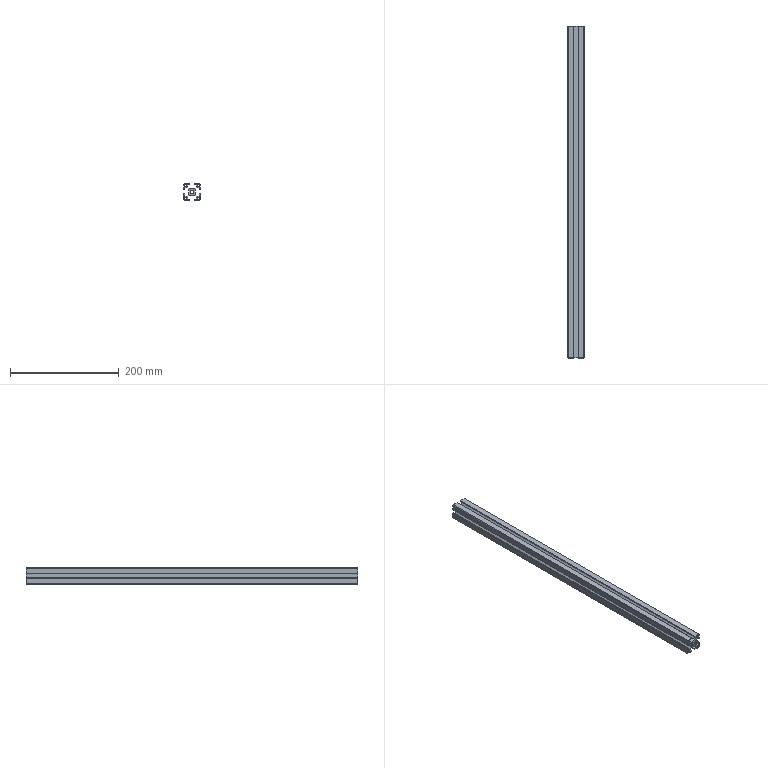Component | SolidWorks | 3030-610-1 | 1 solid | 64 faces | box 30 x 610 x 30 mm | volume 204135 mm3 | plane 46 | cylinder 18 | commonest cylinder face diameters 4.2 x8 0.6 x4 4 x4 6.8 x2
build123d program:
from build123d import *

# Parameters (mm, degrees)
SKETCH1_R           = 2.1
SKETCH1_R_2         = 3.4
BOSS_EXTRUDE1_DEPTH = 610


with BuildPart() as part:
    # Sketch1 → Boss-Extrude1 (new body)
    with BuildSketch(Plane(origin=(0, 0, -100), x_dir=(-1, 0, 0), z_dir=(0, 0, -1))):
        with BuildLine():
            Line((15, 3.8), (15, 13.5))
            ThreePointArc((15, 13.5), (14.823, 14.323), (14.323, 15))
            Line((14.323, 15), (4, 15))
            Line((4, 15), (4, 13))
            Line((4, 13), (8.25, 13))
            Line((8.25, 13), (8.25, 9.664))
            Line((8.25, 9.664), (4.586, 6))
            Line((4.586, 6), (-4.586, 6))
            Line((-4.586, 6), (-8.25, 9.664))
            Line((-8.25, 9.664), (-8.25, 13))
            Line((-8.25, 13), (-4, 13))
            Line((-4, 13), (-4, 15))
            Line((-4, 15), (-14.323, 15))
            ThreePointArc((-14.323, 15), (-14.823, 14.323), (-15, 13.5))
            Line((-15, 13.5), (-15, 3.8))
            ThreePointArc((-15, 3.8), (-14.912, 3.588), (-14.7, 3.5))
            Line((-14.7, 3.5), (-13, 3.5))
            Line((-13, 3.5), (-13, 8.25))
            Line((-13, 8.25), (-9.664, 8.25))
            Line((-9.664, 8.25), (-6, 4.586))
            Line((-6, 4.586), (-6, -4.586))
            Line((-6, -4.586), (-9.664, -8.25))
            Line((-9.664, -8.25), (-13, -8.25))
            Line((-13, -8.25), (-13, -4.5))
            Line((-13, -4.5), (-14.7, -4.5))
            ThreePointArc((-14.7, -4.5), (-14.912, -4.588), (-15, -4.8))
            Line((-15, -4.8), (-15, -13.5))
            ThreePointArc((-15, -13.5), (-14.823, -14.323), (-14.323, -15))
            Line((-14.323, -15), (-4, -15))
            Line((-4, -15), (-4, -13))
            Line((-4, -13), (-8.25, -13))
            Line((-8.25, -13), (-8.25, -9.664))
            Line((-8.25, -9.664), (-4.586, -6))
            Line((-4.586, -6), (4.586, -6))
            Line((4.586, -6), (8.25, -9.664))
            Line((8.25, -9.664), (8.25, -13))
            Line((8.25, -13), (4, -13))
            Line((4, -13), (4, -15))
            Line((4, -15), (14.323, -15))
            ThreePointArc((14.323, -15), (14.823, -14.323), (15, -13.5))
            Line((15, -13.5), (15, -4.8))
            ThreePointArc((15, -4.8), (14.912, -4.588), (14.7, -4.5))
            Line((14.7, -4.5), (13, -4.5))
            Line((13, -4.5), (13, -8.25))
            Line((13, -8.25), (9.664, -8.25))
            Line((9.664, -8.25), (6, -4.586))
            Line((6, -4.586), (6, 4.586))
            Line((6, 4.586), (9.664, 8.25))
            Line((9.664, 8.25), (13, 8.25))
            Line((13, 8.25), (13, 3.5))
            Line((13, 3.5), (14.7, 3.5))
            ThreePointArc((14.7, 3.5), (14.912, 3.588), (15, 3.8))
        make_face()
        with Locations(Location((11.625, 11.625, 0), (0, 0, 180))):
            Circle(SKETCH1_R, mode=Mode.SUBTRACT)
        with Locations(Location((11.625, -11.625, 0), (0, 0, 180))):
            Circle(SKETCH1_R, mode=Mode.SUBTRACT)
        with Locations(Location((0, 0, 0), (0, 0, 180))):
            Circle(SKETCH1_R_2, mode=Mode.SUBTRACT)
        with Locations(Location((-11.625, 11.625, 0), (0, 0, 180))):
            Circle(SKETCH1_R, mode=Mode.SUBTRACT)
        with Locations(Location((-11.625, -11.625, 0), (0, 0, 180))):
            Circle(SKETCH1_R, mode=Mode.SUBTRACT)
    extrude(amount=-BOSS_EXTRUDE1_DEPTH)


solid = part.part

# Placed as in the assembly
solid = solid.moved(Location((-13.047, 112.523, -435), (-90, 0, 0)))